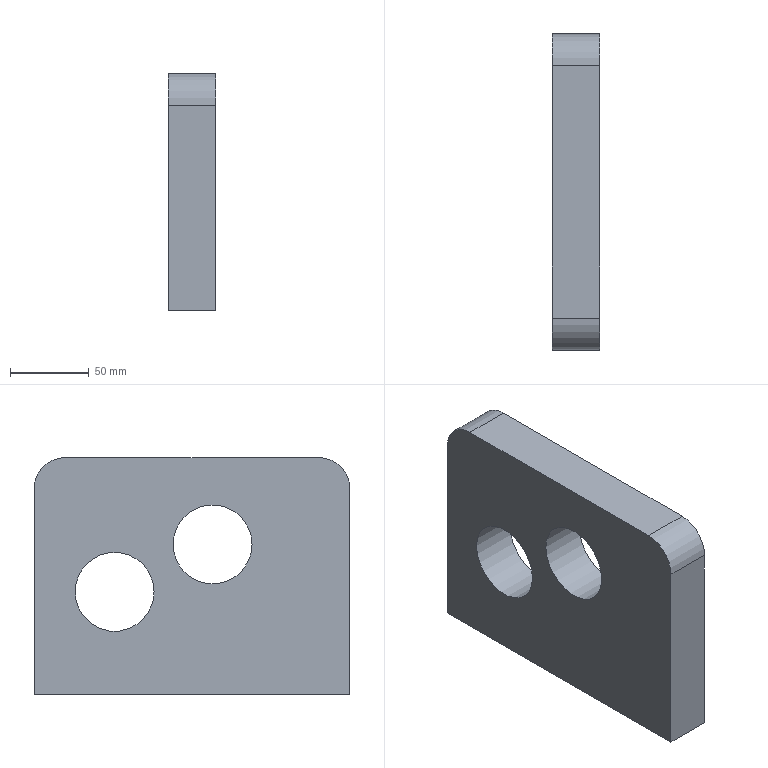Component | NX | TEMPLATE_2 | 1 solid | 16 faces | volume 766710 mm3 | plane 6 | cylinder 6 | cone 4 | commonest cylinder face diameters 50 x2 40 x2 14 x2